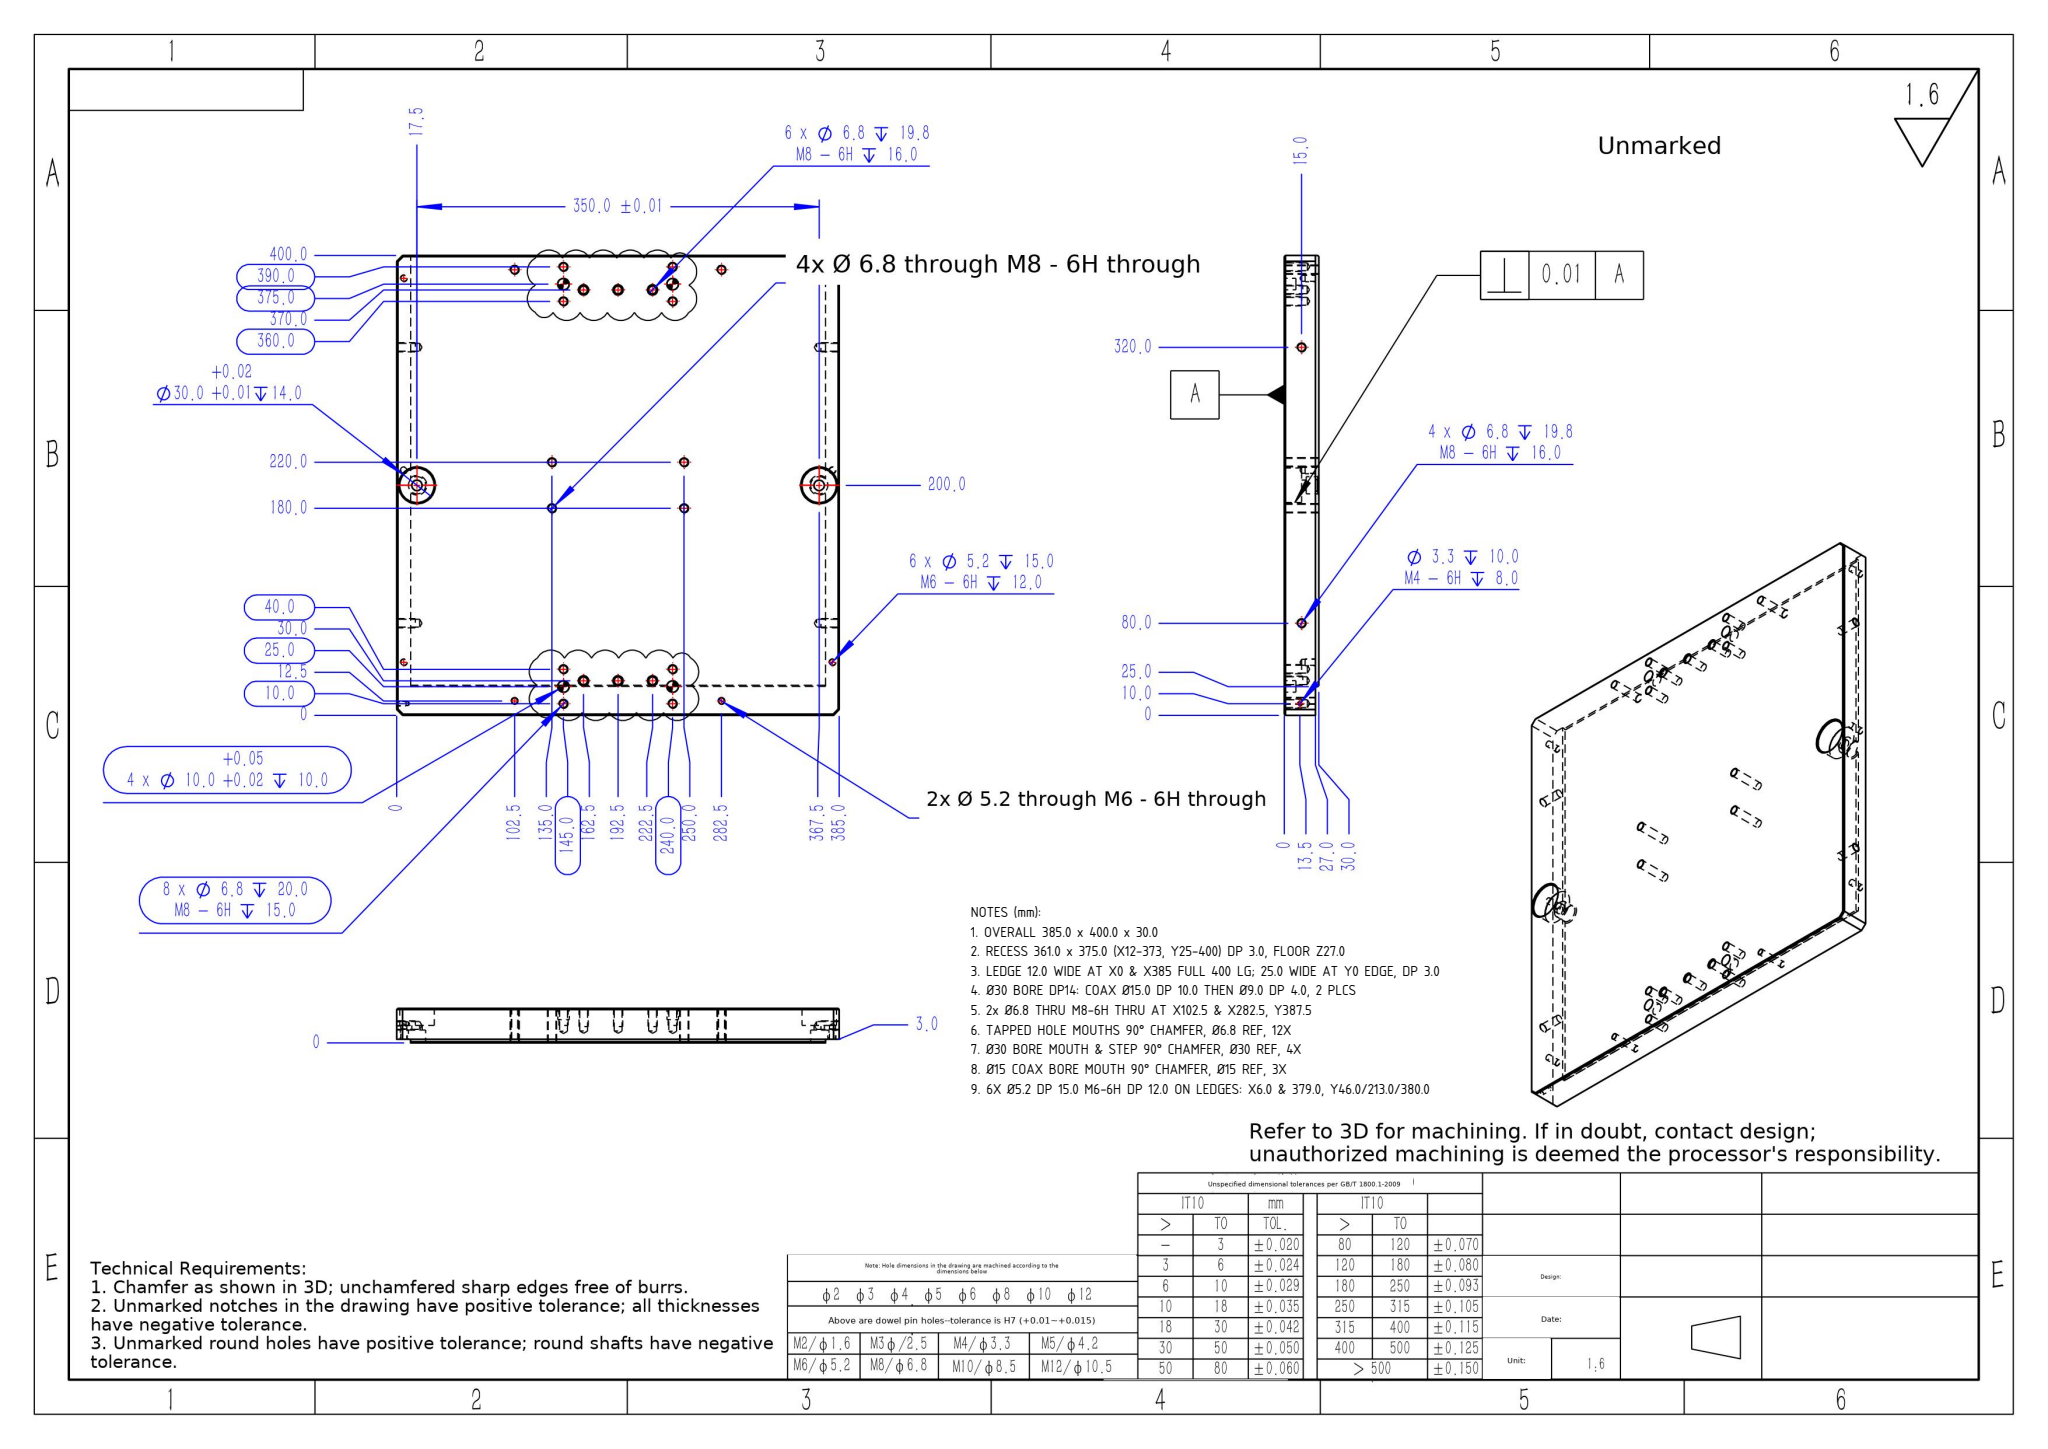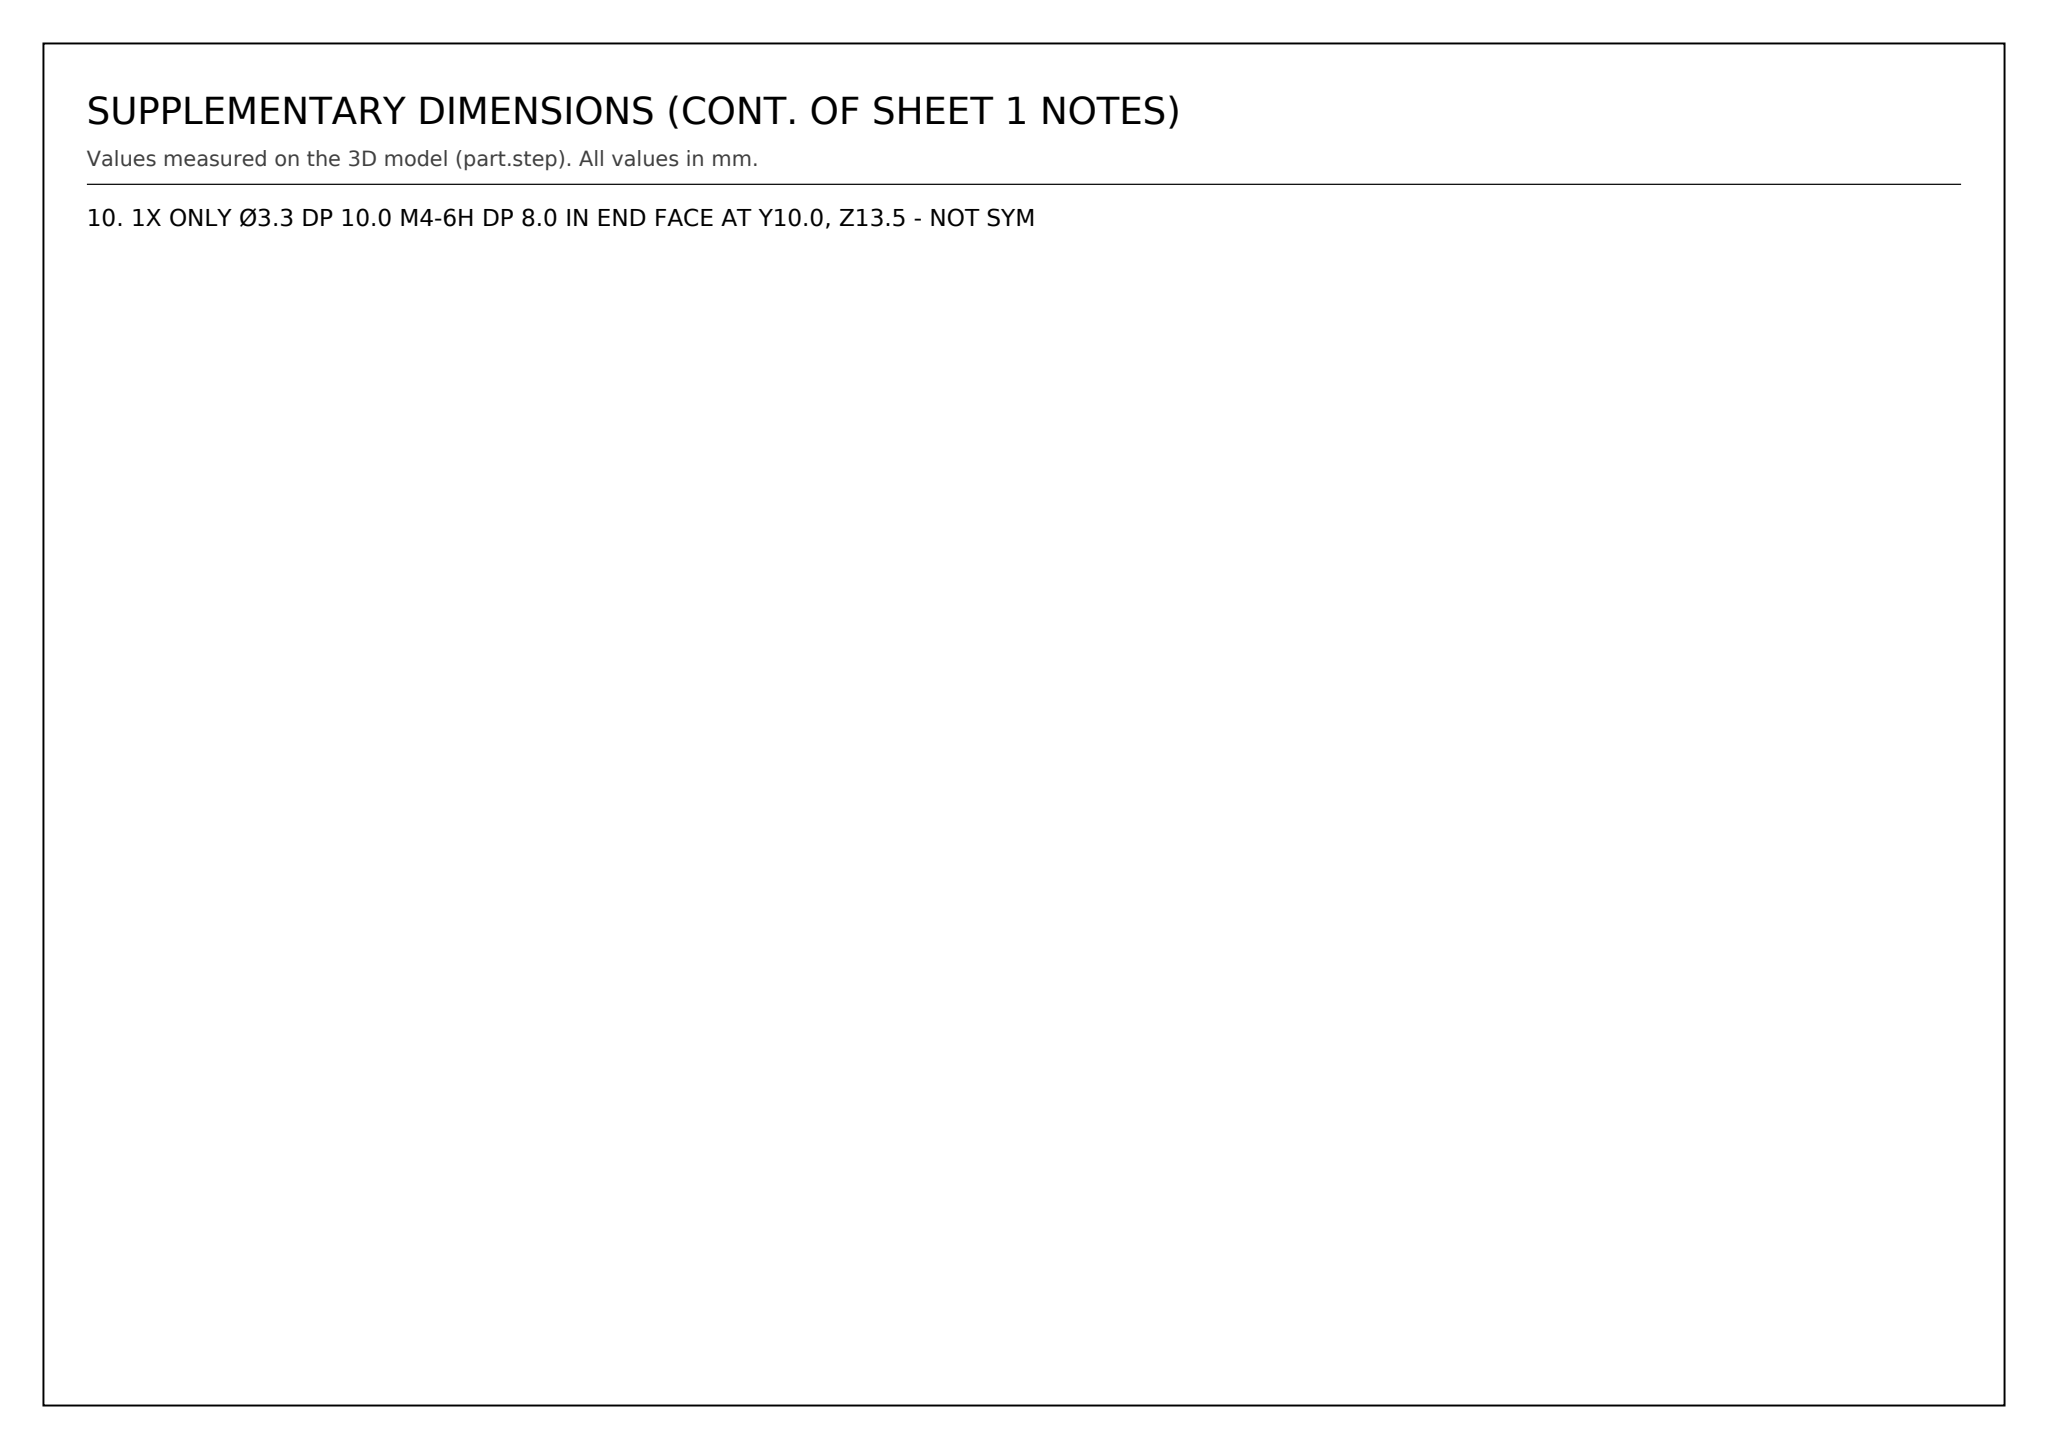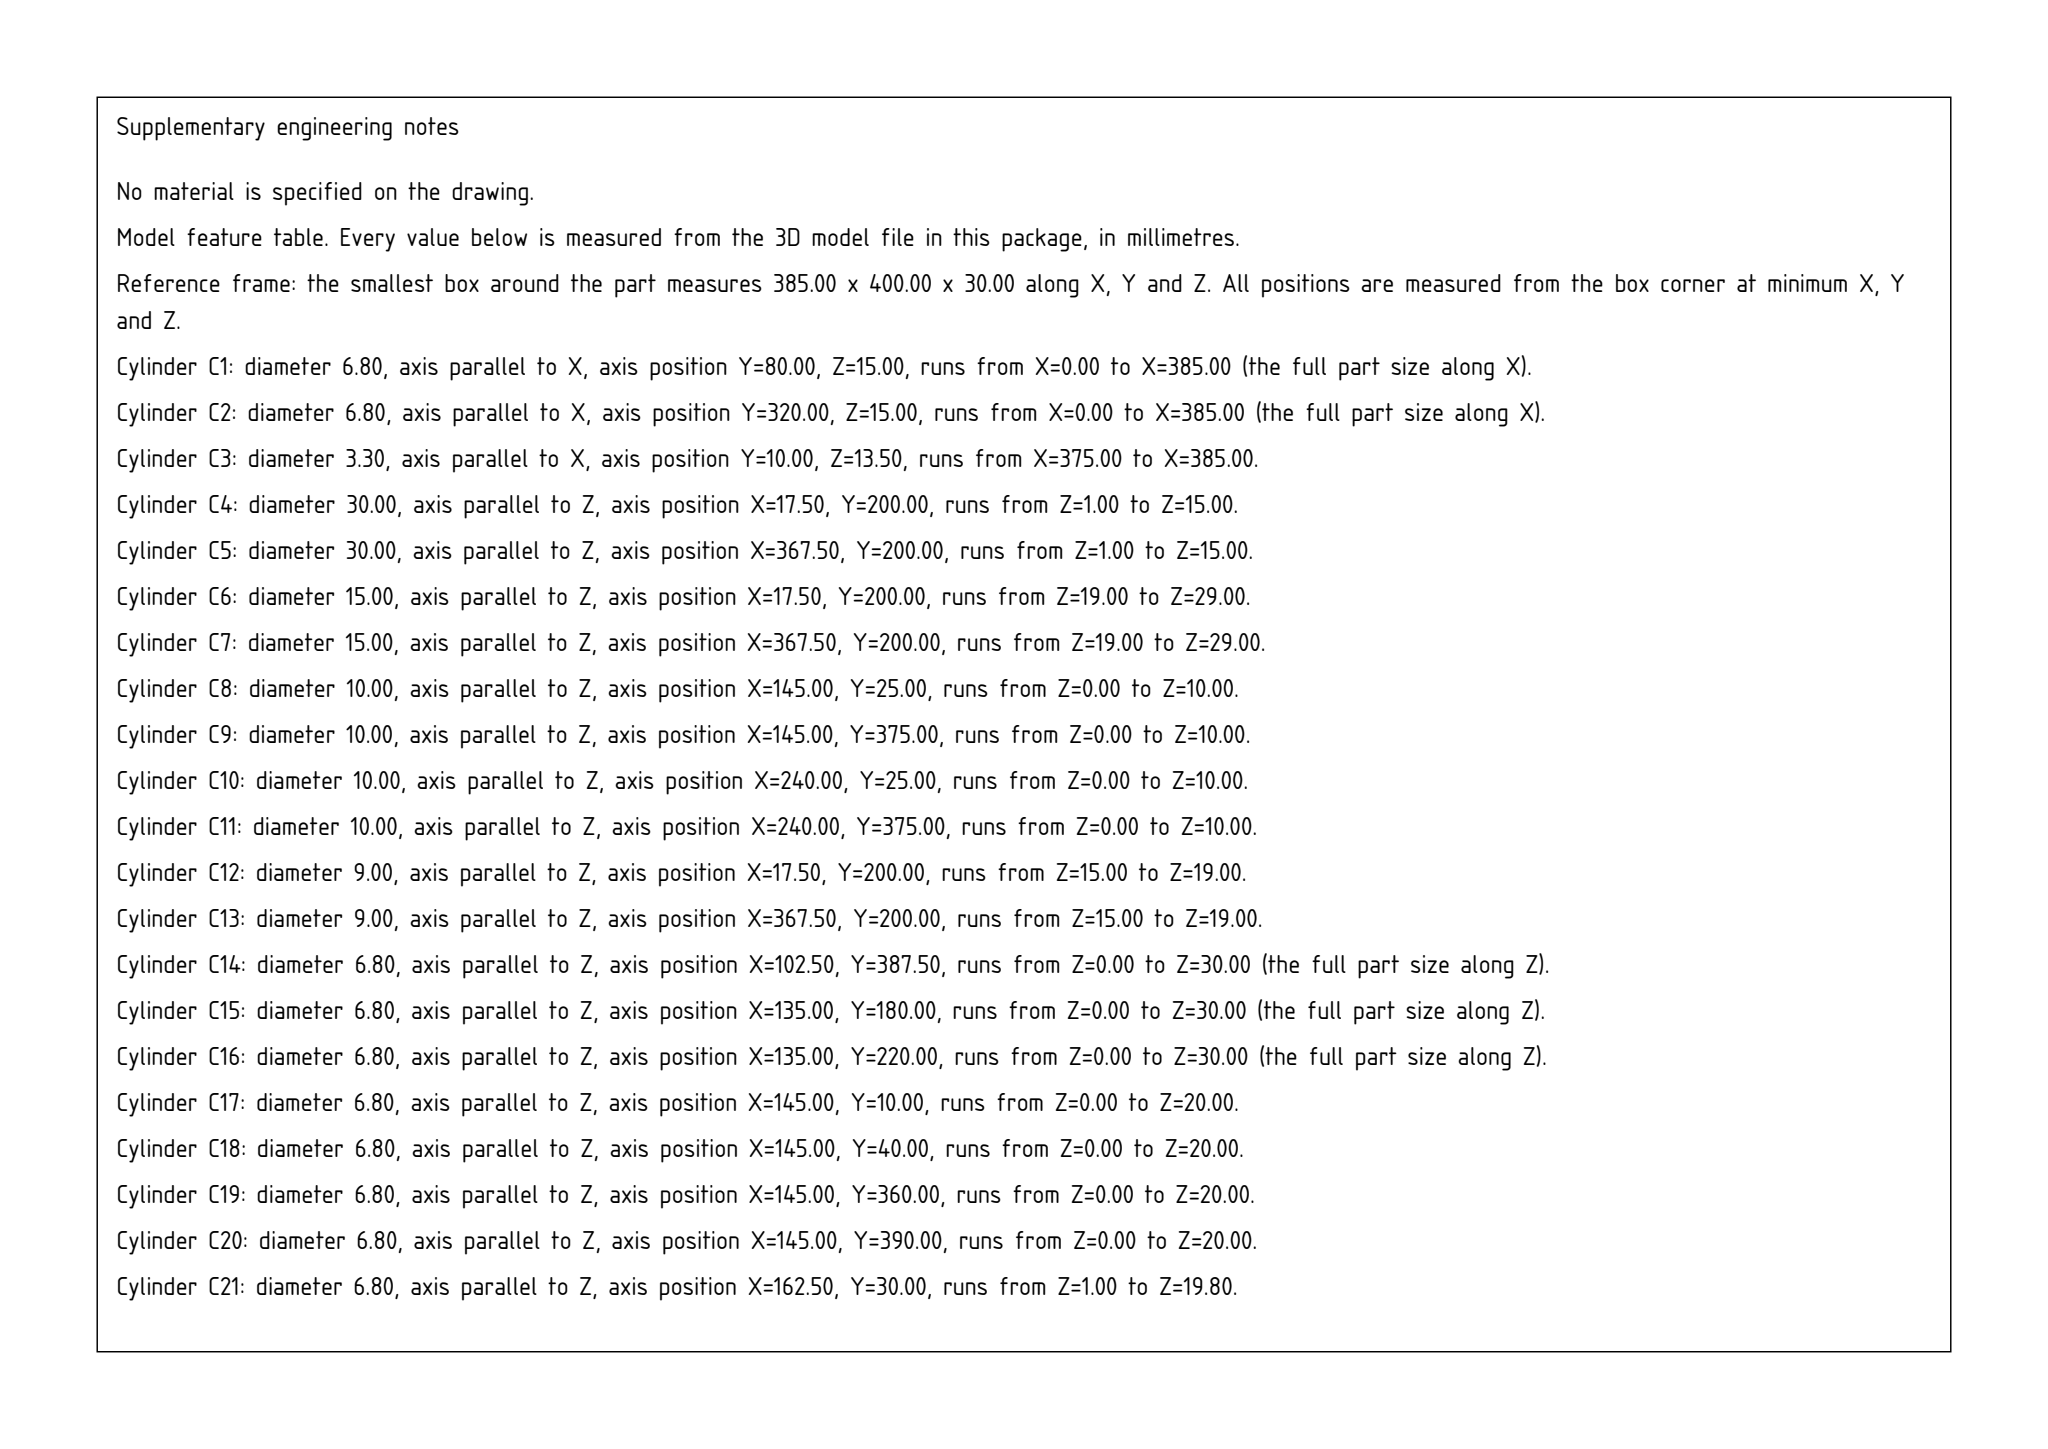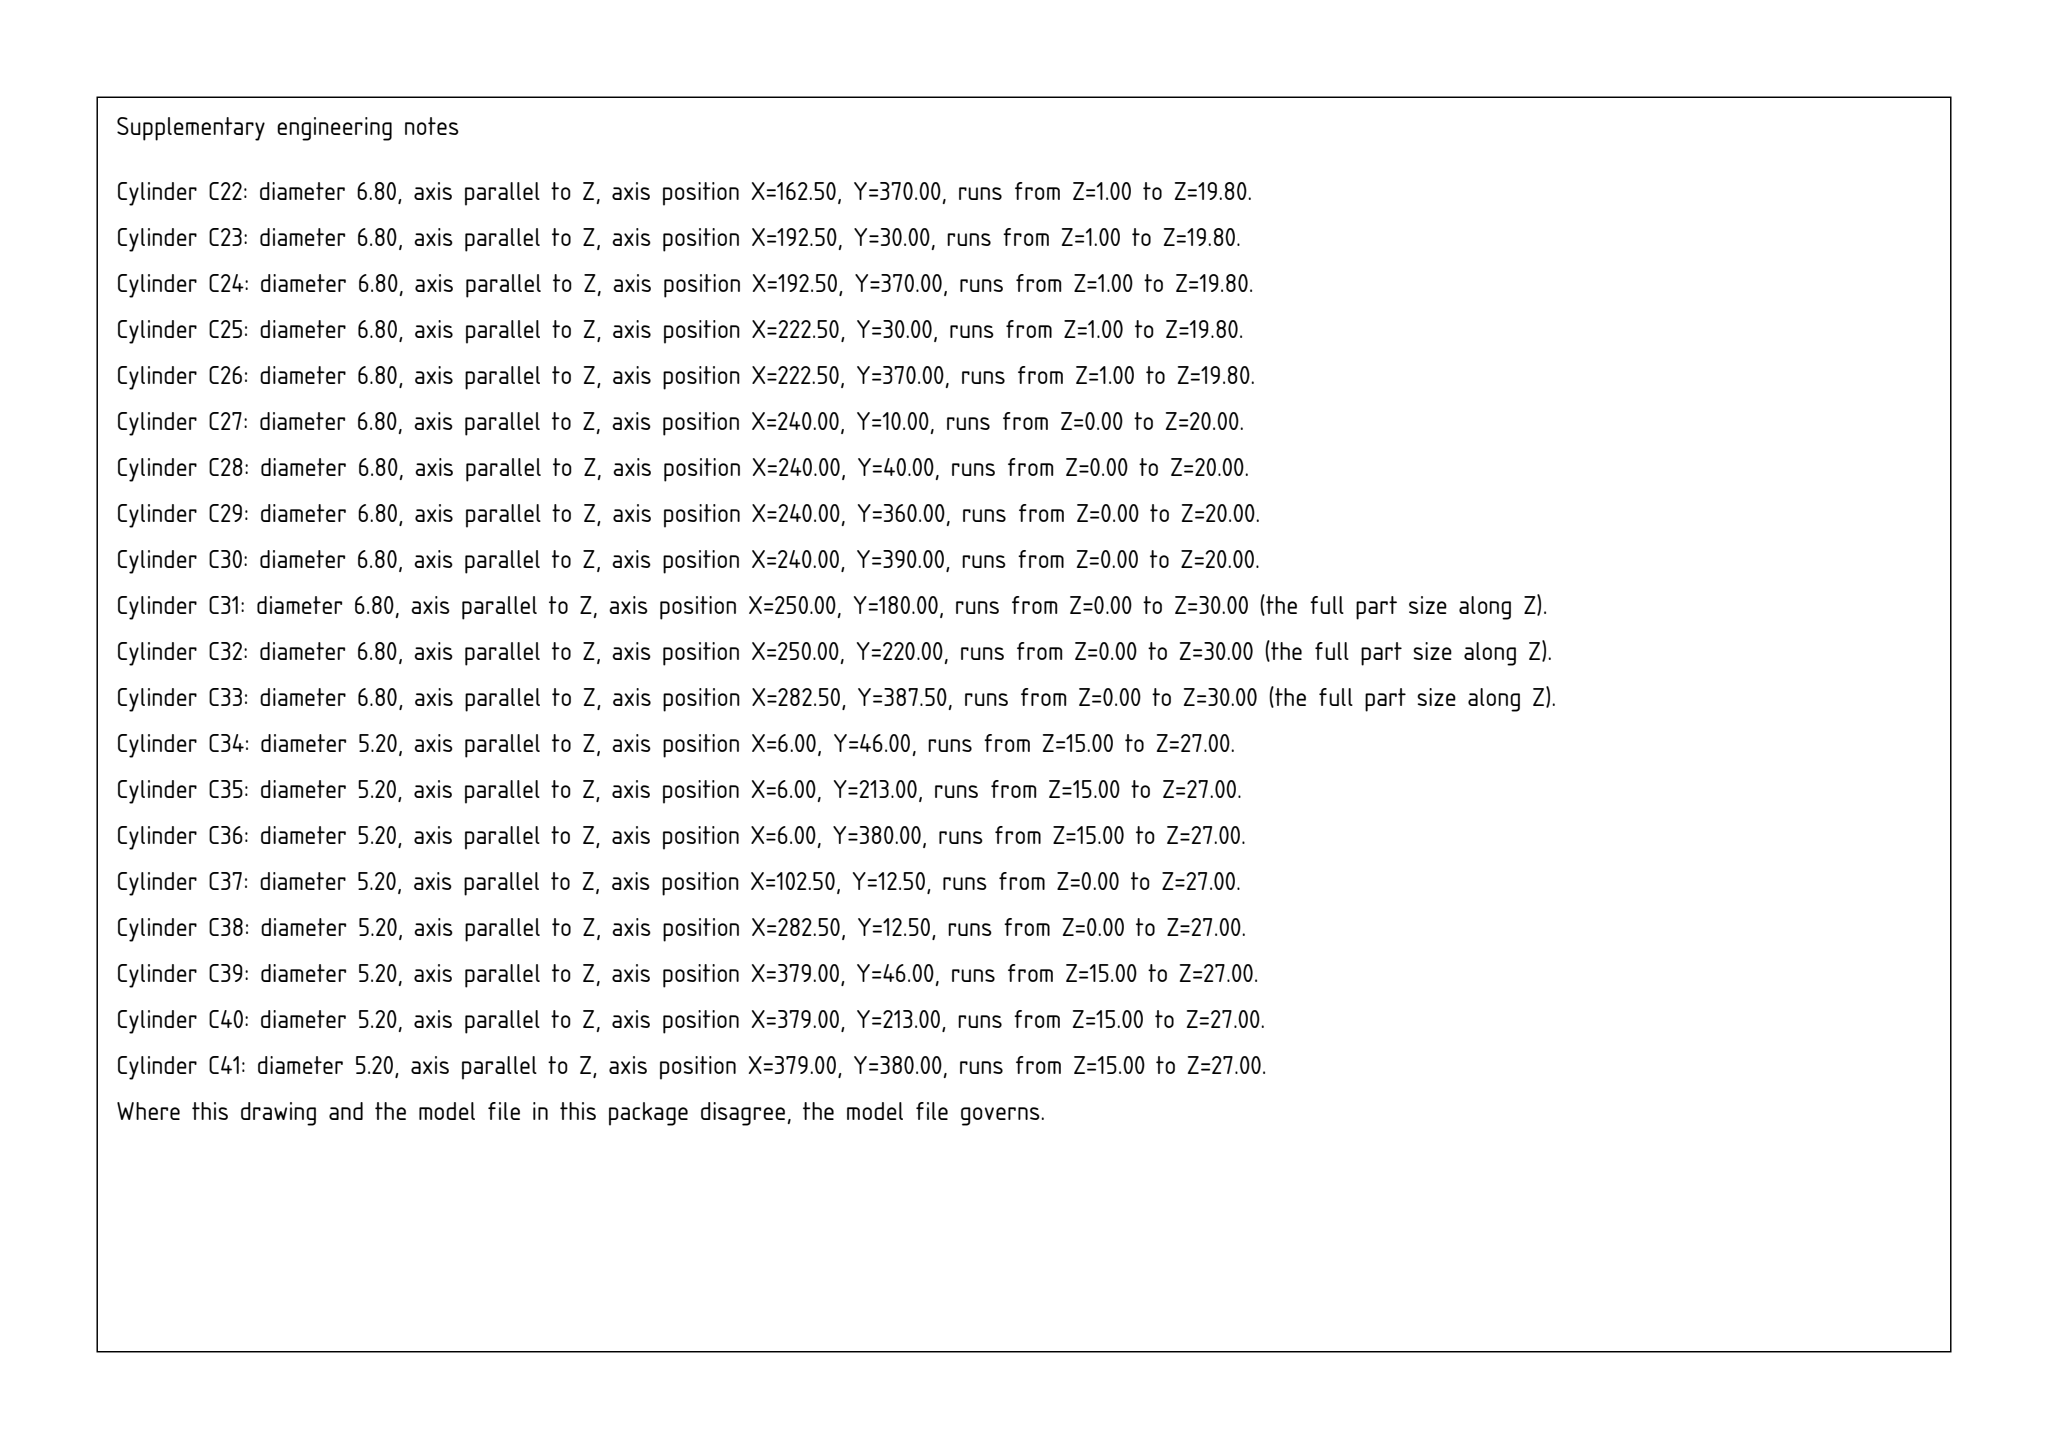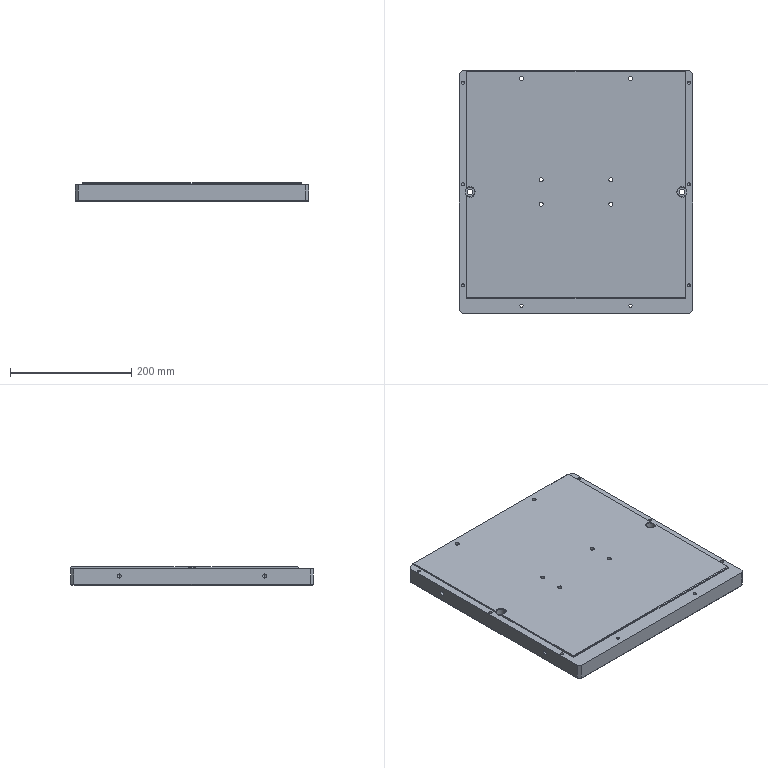Part | SolidWorks | mm | 1 solid | 189 faces | box 385 x 400 x 30 mm | volume 4509958 mm3 | cylinder 86 | cone 69 | plane 34 | commonest cylinder face diameters 6.8 x48 5.2 x16 10 x8 9 x4 15 x4 30 x4 3.3 x2
Drawing notes:
OVERALL 385.0 x 400.0 x 30.0 | from the solid: bbox_xyz [385,400,30]
RECESS 361.0 x 375.0 (X12-373, Y25-400) DP 3.0, FLOOR Z27.0 | from the solid: planes x=12.0/373.0, y=25.0/400.0, floor z=27.0 vs top z=30.0
LEDGE 12.0 WIDE AT X0 & X385 FULL 400 LG; 25.0 WIDE AT Y0 EDGE, DP 3.0 | from the solid: axis planes x=12.0 & x=373.0 (2 each), y=25.0, floor z=27.0, bbox Y=400
Ø30 BORE DP14: COAX Ø15.0 DP 10.0 THEN Ø9.0 DP 4.0, 2 PLCS | from the solid: coax z-cyls Ø30 L14, Ø15 L10, Ø9 L4 at (17.5,200) & (367.5,200); planes z=19, z=15
2x Ø6.8 THRU M8-6H THRU AT X102.5 & X282.5, Y387.5 | from the solid: Ø6.8 z-cyls L=30 (full thk) at (102.5,387.5),(282.5,387.5)
TAPPED HOLE MOUTHS 90° CHAMFER, Ø6.8 REF, 12X | from the solid: cones [90.0, 6.8, 12] on Ø6.8 tap drills
Ø30 BORE MOUTH & STEP 90° CHAMFER, Ø30 REF, 4X | from the solid: cones [90.0, 30.0, 4] at Ø30 DP14 bores (X17.5/367.5, Y200)
Ø15 COAX BORE MOUTH 90° CHAMFER, Ø15 REF, 3X | from the solid: cones [90.0, 15.0, 3] at coax Ø15 DP10 bores
6X Ø5.2 DP 15.0 M6-6H DP 12.0 ON LEDGES: X6.0 & 379.0, Y46.0/213.0/380.0 | from the solid: Ø5.2 z-axis cyls, L=12.0, at (6.0,46.0),(6.0,213.0),(6.0,380.0),(379.0,46.0),(379.0,213.0),(379.0,380.0); ledge faces x=12.0 & x=373.0
1X ONLY Ø3.3 DP 10.0 M4-6H DP 8.0 IN END FACE AT Y10.0, Z13.5 - NOT SYM | from the solid: [3.3,"x",[null,10.0,13.5],10.0,2] = one hole (2 split faces); 118° ref 3.3 count 2 = 1 drill point
build123d program:
from build123d import *

# Parameters (mm, degrees)
SKETCH1_W                                       = 385
SKETCH1_H                                       = 400
BOSS_EXTRUDE1_DEPTH                             = 30
SKETCH4_W                                       = 385
SKETCH4_H                                       = 25
CUT_EXTRUDE1_DEPTH                              = 3
SKETCH5_R                                       = 15
CUT_EXTRUDE2_DEPTH                              = 15
M8_TAPPED_HOLE1_AT_2_COUNT                      = 2
M8_TAPPED_HOLE1_AT_2_PITCH                      = 30
M8_TAPPED_HOLE1_AT_3_COUNT                      = 2
M8_TAPPED_HOLE1_AT_3_PITCH                      = 60
CHAMFER1_SIZE                                   = 5
M8_HEX_SOCKET_HEAD_CAP_SCREW_CBORE1_D           = 9
M8_HEX_SOCKET_HEAD_CAP_SCREW_CBORE1_CBORE_D     = 15
M8_HEX_SOCKET_HEAD_CAP_SCREW_CBORE1_CBORE_DEPTH = 11
M6_TAPPED_HOLE1_D                               = 5.2
M6_TAPPED_HOLE1_DEPTH                           = 15
M6_TAPPED_HOLE1_TIP                             = 1.562
CHAMFER2_SIZE                                   = 1
M8_TAPPED_HOLE3_D                               = 6.8
M4_TAPPED_HOLE1_D                               = 3.3
M4_TAPPED_HOLE1_DEPTH                           = 10
M4_TAPPED_HOLE1_TIP                             = 0.9914
M6_TAPPED_HOLE3_D                               = 5.2
M6_TAPPED_HOLE4_D                               = 5.2
M6_TAPPED_HOLE4_DEPTH                           = 15
M6_TAPPED_HOLE4_TIP                             = 1.562
SKETCH26_W                                      = 12
SKETCH26_H                                      = 375
CUT_EXTRUDE3_DEPTH                              = 3
M8_TAPPED_HOLE4_D                               = 6.8
SIZE_MM_DOWEL_HOLE1_D                           = 10
SIZE_MM_DOWEL_HOLE1_DEPTH                       = 10
M8_TAPPED_HOLE5_D                               = 6.8
M8_TAPPED_HOLE5_DEPTH                           = 20
M8_TAPPED_HOLE5_TIP                             = 2.043


with BuildPart() as part:
    # Sketch1 → Boss-Extrude1 (new body)
    with BuildSketch(Plane.XY):
        Rectangle(SKETCH1_W, SKETCH1_H)
    extrude(amount=BOSS_EXTRUDE1_DEPTH)

    # Sketch4 → Cut-Extrude1 (cut)
    with BuildSketch(Plane.XY.offset(30)):
        with Locations((0, -187.5)):
            Rectangle(SKETCH4_W, SKETCH4_H)
    extrude(amount=-CUT_EXTRUDE1_DEPTH, mode=Mode.SUBTRACT)

    # Sketch5 → Cut-Extrude2 (cut)
    with BuildSketch(Plane(origin=(0, 0, 0), x_dir=(-1, 0, 0), z_dir=(0, 0, -1))):
        with Locations((-175, 0)):
            Circle(SKETCH5_R)
        with Locations((175, 0)):
            Circle(SKETCH5_R)
    extrude(amount=-CUT_EXTRUDE2_DEPTH, mode=Mode.SUBTRACT)

    # Sketch7 → M8 Tapped Hole1 (revolve, cut)
    with BuildSketch(Plane(origin=(-30, 170, 0), x_dir=(0, 1, 0), z_dir=(1, 0, 0))):
        Polygon((0, 0), (0, 21.843), (3.4, 19.8), (3.4, 0), align=None)
    m8_tapped_hole1 = revolve(axis=Axis((-30, 170, -6.35), (0, 0, 1)), mode=Mode.SUBTRACT)

    # M8 Tapped Hole1 at 2: M8 Tapped Hole1 ×2
    with Locations(*[(i * M8_TAPPED_HOLE1_AT_2_PITCH, 0, 0) for i in range(1, M8_TAPPED_HOLE1_AT_2_COUNT)]):
        add(m8_tapped_hole1, mode=Mode.SUBTRACT)

    # M8 Tapped Hole1 at 3: M8 Tapped Hole1 ×2
    with Locations(*[(i * M8_TAPPED_HOLE1_AT_3_PITCH, 0, 0) for i in range(1, M8_TAPPED_HOLE1_AT_3_COUNT)]):
        add(m8_tapped_hole1, mode=Mode.SUBTRACT)

    # Mirror1: M8 Tapped Hole1 across plane
    add(m8_tapped_hole1.mirror(Plane.ZX), mode=Mode.SUBTRACT)

    # Mirror1 copy 1 sketch → Mirror1 copy 1 (revolve, cut)
    with BuildSketch(Plane(origin=(0, -170, 0), x_dir=(0, -1, 0), z_dir=(1, 0, 0))):
        Polygon((0, 0), (0, -21.843), (3.4, -19.8), (3.4, 0), align=None)
    revolve(axis=Axis((0, -170, -6.35), (0, 0, -1)), mode=Mode.SUBTRACT)

    # Mirror1 copy 2 sketch → Mirror1 copy 2 (revolve, cut)
    with BuildSketch(Plane(origin=(30, -170, 0), x_dir=(0, -1, 0), z_dir=(1, 0, 0))):
        Polygon((0, 0), (0, -21.843), (3.4, -19.8), (3.4, 0), align=None)
    revolve(axis=Axis((30, -170, -6.35), (0, 0, -1)), mode=Mode.SUBTRACT)

    # Chamfer1
    chamfer1_edges = [part.edges().sort_by_distance(p)[0] for p in [
        (192.5, -200, 13.5),
        (-192.5, -200, 13.5),
        (-192.5, 200, 15),
        (192.5, 200, 15),
    ]]
    chamfer(chamfer1_edges, length=CHAMFER1_SIZE)

    # M8 Hex Socket Head Cap Screw CBORE1 (through all)
    with Locations(Plane.XY.offset(30)):
        with Locations((175, 0), (-175, 0)):
            CounterBoreHole(M8_HEX_SOCKET_HEAD_CAP_SCREW_CBORE1_D / 2, M8_HEX_SOCKET_HEAD_CAP_SCREW_CBORE1_CBORE_D / 2, M8_HEX_SOCKET_HEAD_CAP_SCREW_CBORE1_CBORE_DEPTH)

    # M6 Tapped Hole1
    with Locations(Plane.XY.offset(30)):
        with Locations((-186.5, -154), (-186.5, 180), (186.5, -154), (186.5, 13), (186.5, 180), (-186.5, 13)):
            Hole(M6_TAPPED_HOLE1_D / 2, depth=M6_TAPPED_HOLE1_DEPTH)
            with Locations((0, 0, -(M6_TAPPED_HOLE1_DEPTH + M6_TAPPED_HOLE1_TIP / 2))):  # 118° drill point
                Cone(0, M6_TAPPED_HOLE1_D / 2, M6_TAPPED_HOLE1_TIP, mode=Mode.SUBTRACT)

    # Sketch13 → M8 Tapped Hole2 (revolve, cut)
    with BuildSketch(Plane(origin=(-192.5, -120, 15), x_dir=(0, 0, 1), z_dir=(0, 1, 0))):
        Polygon((0, 0), (0, 21.843), (3.4, 19.8), (3.4, 0), align=None)
    m8_tapped_hole2 = revolve(axis=Axis((-198.85, -120, 15), (1, 0, 0)), mode=Mode.SUBTRACT)

    # Mirror2: M8 Tapped Hole2 across plane
    add(m8_tapped_hole2.mirror(Plane.ZX), mode=Mode.SUBTRACT)

    # Mirror3: M8 Tapped Hole2 across plane
    add(m8_tapped_hole2.mirror(Plane(origin=(0, 0, 0), x_dir=(0, 0, 1), z_dir=(1, 0, 0))), mode=Mode.SUBTRACT)

    # Mirror3 copy 1 sketch → Mirror3 copy 1 (revolve, cut)
    with BuildSketch(Plane(origin=(192.5, 120, 15), x_dir=(0, 0, 1), z_dir=(0, -1, 0))):
        Polygon((0, 0), (0, 21.843), (3.4, 19.8), (3.4, 0), align=None)
    revolve(axis=Axis((198.85, 120, 15), (-1, 0, 0)), mode=Mode.SUBTRACT)

    # Chamfer2
    chamfer2_edges = [part.edges().sort_by_distance(p)[0] for p in [
        (-192.5, 10, 30),
        (0, 200, 30),
        (190, 197.5, 30),
        (-190, 197.5, 30),
        (-182.5, 0, 30),
        (167.5, 0, 30),
        (192.5, 10, 30),
        (-183.9, 13, 30),
        (189.1, 180, 30),
        (189.1, 13, 30),
        (189.1, -154, 30),
        (-183.9, 180, 30),
        (-183.9, -154, 30),
        (0, -175, 30),
        (190, 0, 0),
        (-160, 0, 0),
        (30, 166.6, 0),
        (0, 166.6, 0),
        (-30, 166.6, 0),
        (30, -166.6, 0),
        (0, -166.6, 0),
        (-30, -166.6, 0),
        (192.5, 0, 0),
        (-192.5, 0, 0),
        (0, 200, 0),
        (0, -200, 0),
        (190, 197.5, 0),
        (-190, 197.5, 0),
        (-190, -197.5, 0),
        (190, -197.5, 0),
    ]]
    chamfer(chamfer2_edges, length=CHAMFER2_SIZE)

    # M8 Tapped Hole3 (through all)
    with Locations(Plane(origin=(0, 0, 0), x_dir=(-1, 0, 0), z_dir=(0, 0, -1))):
        with Locations((57.5, -20), (57.5, 20), (-57.5, 20), (-57.5, -20)):
            Hole(M8_TAPPED_HOLE3_D / 2)

    # M4 Tapped Hole1
    with Locations(Plane(origin=(192.5, 0, 0), x_dir=(0, 0, -1), z_dir=(1, 0, 0))):
        with Locations((-13.5, -190)):
            Hole(M4_TAPPED_HOLE1_D / 2, depth=M4_TAPPED_HOLE1_DEPTH)
            with Locations((0, 0, -(M4_TAPPED_HOLE1_DEPTH + M4_TAPPED_HOLE1_TIP / 2))):  # 118° drill point
                Cone(0, M4_TAPPED_HOLE1_D / 2, M4_TAPPED_HOLE1_TIP, mode=Mode.SUBTRACT)

    # M6 Tapped Hole3 (through all)
    with Locations(Plane.XY.offset(27)):
        with Locations((-90, -187.5), (90, -187.5)):
            Hole(M6_TAPPED_HOLE3_D / 2)

    # M6 Tapped Hole4
    with Locations(Plane.XY.offset(30)):
        with Locations((186.5, -154), (186.5, 13), (186.5, 180), (-186.5, 180), (-186.5, 13), (-186.5, -154)):
            Hole(M6_TAPPED_HOLE4_D / 2, depth=M6_TAPPED_HOLE4_DEPTH)
            with Locations((0, 0, -(M6_TAPPED_HOLE4_DEPTH + M6_TAPPED_HOLE4_TIP / 2))):  # 118° drill point
                Cone(0, M6_TAPPED_HOLE4_D / 2, M6_TAPPED_HOLE4_TIP, mode=Mode.SUBTRACT)

    # Sketch26 → Cut-Extrude3 (cut)
    with BuildSketch(Plane.XY.offset(30)):
        with Locations((-186.5, 12.5)):
            Rectangle(SKETCH26_W, SKETCH26_H)
    cut_extrude3 = extrude(amount=-CUT_EXTRUDE3_DEPTH, mode=Mode.SUBTRACT)

    # Mirror4: Cut-Extrude3 across plane
    add(cut_extrude3.mirror(Plane(origin=(0, 0, 0), x_dir=(0, 0, 1), z_dir=(1, 0, 0))), mode=Mode.SUBTRACT)

    # M8 Tapped Hole4 (through all)
    with Locations(Plane.XY.offset(30)):
        with Locations((-90, 187.5)):
            m8_tapped_hole4 = Hole(M8_TAPPED_HOLE4_D / 2)

    # Mirror5: M8 Tapped Hole4 across plane
    add(m8_tapped_hole4.mirror(Plane(origin=(0, 0, 0), x_dir=(0, 0, 1), z_dir=(1, 0, 0))), mode=Mode.SUBTRACT)

    # Size mm Dowel Hole1
    with Locations(Plane(origin=(0, 0, 0), x_dir=(-1, 0, 0), z_dir=(0, 0, -1))):
        with Locations((47.5, 175), (-47.5, 175), (-47.5, -175), (47.5, -175)):
            Hole(SIZE_MM_DOWEL_HOLE1_D / 2, depth=SIZE_MM_DOWEL_HOLE1_DEPTH)

    # M8 Tapped Hole5
    with Locations(Plane(origin=(0, 0, 0), x_dir=(-1, 0, 0), z_dir=(0, 0, -1))):
        with Locations((-47.5, -190), (-47.5, -160), (47.5, -190), (47.5, -160), (-47.5, 160), (-47.5, 190), (47.5, 160), (47.5, 190)):
            Hole(M8_TAPPED_HOLE5_D / 2, depth=M8_TAPPED_HOLE5_DEPTH)
            with Locations((0, 0, -(M8_TAPPED_HOLE5_DEPTH + M8_TAPPED_HOLE5_TIP / 2))):  # 118° drill point
                Cone(0, M8_TAPPED_HOLE5_D / 2, M8_TAPPED_HOLE5_TIP, mode=Mode.SUBTRACT)


solid = part.part